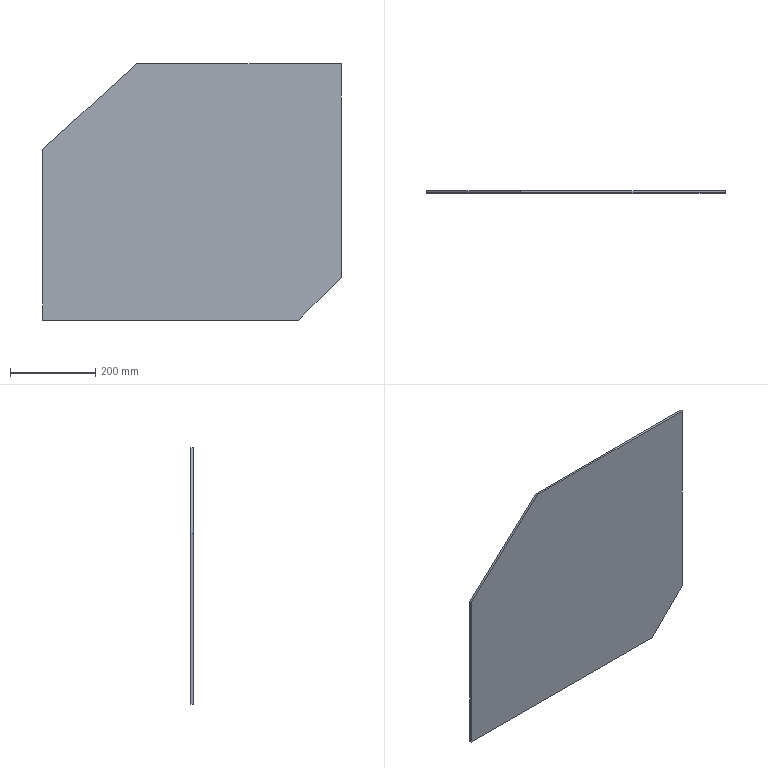Component | NX | CACANBA_2 | 1 solid | 8 faces | box 700 x 5 x 600 mm | volume 1965000 mm3 | plane 8
STEP:
#1=CARTESIAN_POINT('',(0.,0.,0.));
#2=DIRECTION('',(0.,0.,1.));
#3=DIRECTION('',(1.,0.,0.));
#4=AXIS2_PLACEMENT_3D('',#1,#2,#3);
#5=CARTESIAN_POINT('',(-10.,765.233,680.));
#6=VERTEX_POINT('',#5);
#7=CARTESIAN_POINT('',(-10.,765.233,180.));
#8=VERTEX_POINT('',#7);
#9=CARTESIAN_POINT('',(-10.,765.233,680.));
#10=DIRECTION('',(-0.,0.,-1.));
#11=VECTOR('',#10,1.);
#12=LINE('',#9,#11);
#13=CARTESIAN_POINT('',(-10.,770.233,680.));
#14=DIRECTION('',(-1.,0.,0.));
#15=DIRECTION('',(-0.,0.,-1.));
#16=AXIS2_PLACEMENT_3D('',#13,#14,#15);
#17=PLANE('',#16);
#18=CARTESIAN_POINT('',(0.,5.));
#19=DIRECTION('',(1.,0.));
#20=VECTOR('',#19,1.);
#21=LINE('',#18,#20);
#22=(GEOMETRIC_REPRESENTATION_CONTEXT(2)PARAMETRIC_REPRESENTATION_CONTEXT()REPRESENTATION_CONTEXT('',''));
#23=DEFINITIONAL_REPRESENTATION('',(#21),#22);
#24=PCURVE('',#17,#23);
#25=CARTESIAN_POINT('',(-10.,765.233,80.));
#26=DIRECTION('',(0.,1.,0.));
#27=DIRECTION('',(0.,0.,-1.));
#28=AXIS2_PLACEMENT_3D('',#25,#26,#27);
#29=PLANE('',#28);
#30=CARTESIAN_POINT('',(-600.,-0.));
#31=DIRECTION('',(1.,0.));
#32=VECTOR('',#31,1.);
#33=LINE('',#30,#32);
#34=(GEOMETRIC_REPRESENTATION_CONTEXT(2)PARAMETRIC_REPRESENTATION_CONTEXT()REPRESENTATION_CONTEXT('',''));
#35=DEFINITIONAL_REPRESENTATION('',(#33),#34);
#36=PCURVE('',#29,#35);
#37=SURFACE_CURVE('',#12,(#24,#36),.PCURVE_S1.);
#38=EDGE_CURVE('',#6,#8,#37,.T.);
#39=ORIENTED_EDGE('',*,*,#38,.T.);
#40=CARTESIAN_POINT('',(-10.,770.233,180.));
#41=VERTEX_POINT('',#40);
#42=CARTESIAN_POINT('',(-10.,770.233,180.));
#43=DIRECTION('',(0.,-1.,0.));
#44=VECTOR('',#43,1.);
#45=LINE('',#42,#44);
#46=CARTESIAN_POINT('',(500.,0.));
#47=DIRECTION('',(0.,1.));
#48=VECTOR('',#47,1.);
#49=LINE('',#46,#48);
#50=(GEOMETRIC_REPRESENTATION_CONTEXT(2)PARAMETRIC_REPRESENTATION_CONTEXT()REPRESENTATION_CONTEXT('',''));
#51=DEFINITIONAL_REPRESENTATION('',(#49),#50);
#52=PCURVE('',#17,#51);
#53=CARTESIAN_POINT('',(-10.,770.233,180.));
#54=DIRECTION('',(-0.7071,0.,0.7071));
#55=DIRECTION('',(-0.7071,0.,-0.7071));
#56=AXIS2_PLACEMENT_3D('',#53,#54,#55);
#57=PLANE('',#56);
#58=CARTESIAN_POINT('',(0.,0.));
#59=DIRECTION('',(0.,1.));
#60=VECTOR('',#59,1.);
#61=LINE('',#58,#60);
#62=(GEOMETRIC_REPRESENTATION_CONTEXT(2)PARAMETRIC_REPRESENTATION_CONTEXT()REPRESENTATION_CONTEXT('',''));
#63=DEFINITIONAL_REPRESENTATION('',(#61),#62);
#64=PCURVE('',#57,#63);
#65=SURFACE_CURVE('',#45,(#52,#64),.PCURVE_S1.);
#66=EDGE_CURVE('',#41,#8,#65,.T.);
#67=ORIENTED_EDGE('',*,*,#66,.F.);
#68=CARTESIAN_POINT('',(-10.,770.233,680.));
#69=VERTEX_POINT('',#68);
#70=CARTESIAN_POINT('',(-10.,770.233,680.));
#71=DIRECTION('',(-0.,0.,-1.));
#72=VECTOR('',#71,1.);
#73=LINE('',#70,#72);
#74=CARTESIAN_POINT('',(0.,0.));
#75=DIRECTION('',(1.,0.));
#76=VECTOR('',#75,1.);
#77=LINE('',#74,#76);
#78=(GEOMETRIC_REPRESENTATION_CONTEXT(2)PARAMETRIC_REPRESENTATION_CONTEXT()REPRESENTATION_CONTEXT('',''));
#79=DEFINITIONAL_REPRESENTATION('',(#77),#78);
#80=PCURVE('',#17,#79);
#81=CARTESIAN_POINT('',(-10.,770.233,80.));
#82=DIRECTION('',(0.,1.,0.));
#83=DIRECTION('',(0.,0.,-1.));
#84=AXIS2_PLACEMENT_3D('',#81,#82,#83);
#85=PLANE('',#84);
#86=CARTESIAN_POINT('',(-600.,-0.));
#87=DIRECTION('',(1.,0.));
#88=VECTOR('',#87,1.);
#89=LINE('',#86,#88);
#90=(GEOMETRIC_REPRESENTATION_CONTEXT(2)PARAMETRIC_REPRESENTATION_CONTEXT()REPRESENTATION_CONTEXT('',''));
#91=DEFINITIONAL_REPRESENTATION('',(#89),#90);
#92=PCURVE('',#85,#91);
#93=SURFACE_CURVE('',#73,(#80,#92),.PCURVE_S1.);
#94=EDGE_CURVE('',#69,#41,#93,.T.);
#95=ORIENTED_EDGE('',*,*,#94,.F.);
#96=CARTESIAN_POINT('',(-10.,770.233,680.));
#97=DIRECTION('',(0.,-1.,0.));
#98=VECTOR('',#97,1.);
#99=LINE('',#96,#98);
#100=CARTESIAN_POINT('',(0.,0.));
#101=DIRECTION('',(0.,1.));
#102=VECTOR('',#101,1.);
#103=LINE('',#100,#102);
#104=(GEOMETRIC_REPRESENTATION_CONTEXT(2)PARAMETRIC_REPRESENTATION_CONTEXT()REPRESENTATION_CONTEXT('',''));
#105=DEFINITIONAL_REPRESENTATION('',(#103),#104);
#106=PCURVE('',#17,#105);
#107=CARTESIAN_POINT('',(-490.,770.233,680.));
#108=DIRECTION('',(-0.,0.,-1.));
#109=DIRECTION('',(1.,0.,-0.));
#110=AXIS2_PLACEMENT_3D('',#107,#108,#109);
#111=PLANE('',#110);
#112=CARTESIAN_POINT('',(480.,0.));
#113=DIRECTION('',(0.,1.));
#114=VECTOR('',#113,1.);
#115=LINE('',#112,#114);
#116=(GEOMETRIC_REPRESENTATION_CONTEXT(2)PARAMETRIC_REPRESENTATION_CONTEXT()REPRESENTATION_CONTEXT('',''));
#117=DEFINITIONAL_REPRESENTATION('',(#115),#116);
#118=PCURVE('',#111,#117);
#119=SURFACE_CURVE('',#99,(#106,#118),.PCURVE_S1.);
#120=EDGE_CURVE('',#69,#6,#119,.T.);
#121=ORIENTED_EDGE('',*,*,#120,.T.);
#122=EDGE_LOOP('',(#39,#67,#95,#121));
#123=FACE_BOUND('',#122,.T.);
#124=ADVANCED_FACE('',(#123),#17,.F.);
#125=CARTESIAN_POINT('',(-110.,765.233,80.));
#126=VERTEX_POINT('',#125);
#127=CARTESIAN_POINT('',(-10.,765.233,180.));
#128=DIRECTION('',(-0.7071,0.,-0.7071));
#129=VECTOR('',#128,1.);
#130=LINE('',#127,#129);
#131=CARTESIAN_POINT('',(0.,5.));
#132=DIRECTION('',(1.,0.));
#133=VECTOR('',#132,1.);
#134=LINE('',#131,#133);
#135=(GEOMETRIC_REPRESENTATION_CONTEXT(2)PARAMETRIC_REPRESENTATION_CONTEXT()REPRESENTATION_CONTEXT('',''));
#136=DEFINITIONAL_REPRESENTATION('',(#134),#135);
#137=PCURVE('',#57,#136);
#138=CARTESIAN_POINT('',(-100.,0.));
#139=DIRECTION('',(0.7071,0.7071));
#140=VECTOR('',#139,1.);
#141=LINE('',#138,#140);
#142=(GEOMETRIC_REPRESENTATION_CONTEXT(2)PARAMETRIC_REPRESENTATION_CONTEXT()REPRESENTATION_CONTEXT('',''));
#143=DEFINITIONAL_REPRESENTATION('',(#141),#142);
#144=PCURVE('',#29,#143);
#145=SURFACE_CURVE('',#130,(#137,#144),.PCURVE_S1.);
#146=EDGE_CURVE('',#8,#126,#145,.T.);
#147=ORIENTED_EDGE('',*,*,#146,.T.);
#148=CARTESIAN_POINT('',(-110.,770.233,80.));
#149=VERTEX_POINT('',#148);
#150=CARTESIAN_POINT('',(-110.,770.233,80.));
#151=DIRECTION('',(0.,-1.,0.));
#152=VECTOR('',#151,1.);
#153=LINE('',#150,#152);
#154=CARTESIAN_POINT('',(141.421,0.));
#155=DIRECTION('',(0.,1.));
#156=VECTOR('',#155,1.);
#157=LINE('',#154,#156);
#158=(GEOMETRIC_REPRESENTATION_CONTEXT(2)PARAMETRIC_REPRESENTATION_CONTEXT()REPRESENTATION_CONTEXT('',''));
#159=DEFINITIONAL_REPRESENTATION('',(#157),#158);
#160=PCURVE('',#57,#159);
#161=CARTESIAN_POINT('',(-110.,770.233,80.));
#162=DIRECTION('',(0.,0.,1.));
#163=DIRECTION('',(-1.,0.,0.));
#164=AXIS2_PLACEMENT_3D('',#161,#162,#163);
#165=PLANE('',#164);
#166=CARTESIAN_POINT('',(0.,0.));
#167=DIRECTION('',(0.,1.));
#168=VECTOR('',#167,1.);
#169=LINE('',#166,#168);
#170=(GEOMETRIC_REPRESENTATION_CONTEXT(2)PARAMETRIC_REPRESENTATION_CONTEXT()REPRESENTATION_CONTEXT('',''));
#171=DEFINITIONAL_REPRESENTATION('',(#169),#170);
#172=PCURVE('',#165,#171);
#173=SURFACE_CURVE('',#153,(#160,#172),.PCURVE_S1.);
#174=EDGE_CURVE('',#149,#126,#173,.T.);
#175=ORIENTED_EDGE('',*,*,#174,.F.);
#176=CARTESIAN_POINT('',(-10.,770.233,180.));
#177=DIRECTION('',(-0.7071,0.,-0.7071));
#178=VECTOR('',#177,1.);
#179=LINE('',#176,#178);
#180=CARTESIAN_POINT('',(0.,0.));
#181=DIRECTION('',(1.,0.));
#182=VECTOR('',#181,1.);
#183=LINE('',#180,#182);
#184=(GEOMETRIC_REPRESENTATION_CONTEXT(2)PARAMETRIC_REPRESENTATION_CONTEXT()REPRESENTATION_CONTEXT('',''));
#185=DEFINITIONAL_REPRESENTATION('',(#183),#184);
#186=PCURVE('',#57,#185);
#187=CARTESIAN_POINT('',(-100.,0.));
#188=DIRECTION('',(0.7071,0.7071));
#189=VECTOR('',#188,1.);
#190=LINE('',#187,#189);
#191=(GEOMETRIC_REPRESENTATION_CONTEXT(2)PARAMETRIC_REPRESENTATION_CONTEXT()REPRESENTATION_CONTEXT('',''));
#192=DEFINITIONAL_REPRESENTATION('',(#190),#191);
#193=PCURVE('',#85,#192);
#194=SURFACE_CURVE('',#179,(#186,#193),.PCURVE_S1.);
#195=EDGE_CURVE('',#41,#149,#194,.T.);
#196=ORIENTED_EDGE('',*,*,#195,.F.);
#197=ORIENTED_EDGE('',*,*,#66,.T.);
#198=EDGE_LOOP('',(#147,#175,#196,#197));
#199=FACE_BOUND('',#198,.T.);
#200=ADVANCED_FACE('',(#199),#57,.F.);
#201=CARTESIAN_POINT('',(-710.,765.233,80.));
#202=VERTEX_POINT('',#201);
#203=CARTESIAN_POINT('',(-110.,765.233,80.));
#204=DIRECTION('',(-1.,0.,0.));
#205=VECTOR('',#204,1.);
#206=LINE('',#203,#205);
#207=CARTESIAN_POINT('',(0.,5.));
#208=DIRECTION('',(1.,0.));
#209=VECTOR('',#208,1.);
#210=LINE('',#207,#209);
#211=(GEOMETRIC_REPRESENTATION_CONTEXT(2)PARAMETRIC_REPRESENTATION_CONTEXT()REPRESENTATION_CONTEXT('',''));
#212=DEFINITIONAL_REPRESENTATION('',(#210),#211);
#213=PCURVE('',#165,#212);
#214=CARTESIAN_POINT('',(0.,100.));
#215=DIRECTION('',(-0.,1.));
#216=VECTOR('',#215,1.);
#217=LINE('',#214,#216);
#218=(GEOMETRIC_REPRESENTATION_CONTEXT(2)PARAMETRIC_REPRESENTATION_CONTEXT()REPRESENTATION_CONTEXT('',''));
#219=DEFINITIONAL_REPRESENTATION('',(#217),#218);
#220=PCURVE('',#29,#219);
#221=SURFACE_CURVE('',#206,(#213,#220),.PCURVE_S1.);
#222=EDGE_CURVE('',#126,#202,#221,.T.);
#223=ORIENTED_EDGE('',*,*,#222,.T.);
#224=CARTESIAN_POINT('',(-710.,770.233,80.));
#225=VERTEX_POINT('',#224);
#226=CARTESIAN_POINT('',(-710.,770.233,80.));
#227=DIRECTION('',(0.,-1.,0.));
#228=VECTOR('',#227,1.);
#229=LINE('',#226,#228);
#230=CARTESIAN_POINT('',(600.,0.));
#231=DIRECTION('',(0.,1.));
#232=VECTOR('',#231,1.);
#233=LINE('',#230,#232);
#234=(GEOMETRIC_REPRESENTATION_CONTEXT(2)PARAMETRIC_REPRESENTATION_CONTEXT()REPRESENTATION_CONTEXT('',''));
#235=DEFINITIONAL_REPRESENTATION('',(#233),#234);
#236=PCURVE('',#165,#235);
#237=CARTESIAN_POINT('',(-710.,770.233,80.));
#238=DIRECTION('',(1.,0.,-0.));
#239=DIRECTION('',(0.,0.,1.));
#240=AXIS2_PLACEMENT_3D('',#237,#238,#239);
#241=PLANE('',#240);
#242=CARTESIAN_POINT('',(0.,0.));
#243=DIRECTION('',(0.,1.));
#244=VECTOR('',#243,1.);
#245=LINE('',#242,#244);
#246=(GEOMETRIC_REPRESENTATION_CONTEXT(2)PARAMETRIC_REPRESENTATION_CONTEXT()REPRESENTATION_CONTEXT('',''));
#247=DEFINITIONAL_REPRESENTATION('',(#245),#246);
#248=PCURVE('',#241,#247);
#249=SURFACE_CURVE('',#229,(#236,#248),.PCURVE_S1.);
#250=EDGE_CURVE('',#225,#202,#249,.T.);
#251=ORIENTED_EDGE('',*,*,#250,.F.);
#252=CARTESIAN_POINT('',(-110.,770.233,80.));
#253=DIRECTION('',(-1.,0.,0.));
#254=VECTOR('',#253,1.);
#255=LINE('',#252,#254);
#256=CARTESIAN_POINT('',(0.,0.));
#257=DIRECTION('',(1.,0.));
#258=VECTOR('',#257,1.);
#259=LINE('',#256,#258);
#260=(GEOMETRIC_REPRESENTATION_CONTEXT(2)PARAMETRIC_REPRESENTATION_CONTEXT()REPRESENTATION_CONTEXT('',''));
#261=DEFINITIONAL_REPRESENTATION('',(#259),#260);
#262=PCURVE('',#165,#261);
#263=CARTESIAN_POINT('',(0.,100.));
#264=DIRECTION('',(-0.,1.));
#265=VECTOR('',#264,1.);
#266=LINE('',#263,#265);
#267=(GEOMETRIC_REPRESENTATION_CONTEXT(2)PARAMETRIC_REPRESENTATION_CONTEXT()REPRESENTATION_CONTEXT('',''));
#268=DEFINITIONAL_REPRESENTATION('',(#266),#267);
#269=PCURVE('',#85,#268);
#270=SURFACE_CURVE('',#255,(#262,#269),.PCURVE_S1.);
#271=EDGE_CURVE('',#149,#225,#270,.T.);
#272=ORIENTED_EDGE('',*,*,#271,.F.);
#273=ORIENTED_EDGE('',*,*,#174,.T.);
#274=EDGE_LOOP('',(#223,#251,#272,#273));
#275=FACE_BOUND('',#274,.T.);
#276=ADVANCED_FACE('',(#275),#165,.F.);
#277=CARTESIAN_POINT('',(-710.,765.233,480.));
#278=VERTEX_POINT('',#277);
#279=CARTESIAN_POINT('',(-710.,765.233,80.));
#280=DIRECTION('',(0.,0.,1.));
#281=VECTOR('',#280,1.);
#282=LINE('',#279,#281);
#283=CARTESIAN_POINT('',(0.,5.));
#284=DIRECTION('',(1.,0.));
#285=VECTOR('',#284,1.);
#286=LINE('',#283,#285);
#287=(GEOMETRIC_REPRESENTATION_CONTEXT(2)PARAMETRIC_REPRESENTATION_CONTEXT()REPRESENTATION_CONTEXT('',''));
#288=DEFINITIONAL_REPRESENTATION('',(#286),#287);
#289=PCURVE('',#241,#288);
#290=CARTESIAN_POINT('',(-0.,700.));
#291=DIRECTION('',(-1.,-0.));
#292=VECTOR('',#291,1.);
#293=LINE('',#290,#292);
#294=(GEOMETRIC_REPRESENTATION_CONTEXT(2)PARAMETRIC_REPRESENTATION_CONTEXT()REPRESENTATION_CONTEXT('',''));
#295=DEFINITIONAL_REPRESENTATION('',(#293),#294);
#296=PCURVE('',#29,#295);
#297=SURFACE_CURVE('',#282,(#289,#296),.PCURVE_S1.);
#298=EDGE_CURVE('',#202,#278,#297,.T.);
#299=ORIENTED_EDGE('',*,*,#298,.T.);
#300=CARTESIAN_POINT('',(-710.,770.233,480.));
#301=VERTEX_POINT('',#300);
#302=CARTESIAN_POINT('',(-710.,770.233,480.));
#303=DIRECTION('',(0.,-1.,0.));
#304=VECTOR('',#303,1.);
#305=LINE('',#302,#304);
#306=CARTESIAN_POINT('',(400.,0.));
#307=DIRECTION('',(0.,1.));
#308=VECTOR('',#307,1.);
#309=LINE('',#306,#308);
#310=(GEOMETRIC_REPRESENTATION_CONTEXT(2)PARAMETRIC_REPRESENTATION_CONTEXT()REPRESENTATION_CONTEXT('',''));
#311=DEFINITIONAL_REPRESENTATION('',(#309),#310);
#312=PCURVE('',#241,#311);
#313=CARTESIAN_POINT('',(-710.,770.233,480.));
#314=DIRECTION('',(0.6727,0.,-0.7399));
#315=DIRECTION('',(0.7399,0.,0.6727));
#316=AXIS2_PLACEMENT_3D('',#313,#314,#315);
#317=PLANE('',#316);
#318=CARTESIAN_POINT('',(0.,0.));
#319=DIRECTION('',(0.,1.));
#320=VECTOR('',#319,1.);
#321=LINE('',#318,#320);
#322=(GEOMETRIC_REPRESENTATION_CONTEXT(2)PARAMETRIC_REPRESENTATION_CONTEXT()REPRESENTATION_CONTEXT('',''));
#323=DEFINITIONAL_REPRESENTATION('',(#321),#322);
#324=PCURVE('',#317,#323);
#325=SURFACE_CURVE('',#305,(#312,#324),.PCURVE_S1.);
#326=EDGE_CURVE('',#301,#278,#325,.T.);
#327=ORIENTED_EDGE('',*,*,#326,.F.);
#328=CARTESIAN_POINT('',(-710.,770.233,80.));
#329=DIRECTION('',(0.,0.,1.));
#330=VECTOR('',#329,1.);
#331=LINE('',#328,#330);
#332=CARTESIAN_POINT('',(0.,0.));
#333=DIRECTION('',(1.,0.));
#334=VECTOR('',#333,1.);
#335=LINE('',#332,#334);
#336=(GEOMETRIC_REPRESENTATION_CONTEXT(2)PARAMETRIC_REPRESENTATION_CONTEXT()REPRESENTATION_CONTEXT('',''));
#337=DEFINITIONAL_REPRESENTATION('',(#335),#336);
#338=PCURVE('',#241,#337);
#339=CARTESIAN_POINT('',(-0.,700.));
#340=DIRECTION('',(-1.,-0.));
#341=VECTOR('',#340,1.);
#342=LINE('',#339,#341);
#343=(GEOMETRIC_REPRESENTATION_CONTEXT(2)PARAMETRIC_REPRESENTATION_CONTEXT()REPRESENTATION_CONTEXT('',''));
#344=DEFINITIONAL_REPRESENTATION('',(#342),#343);
#345=PCURVE('',#85,#344);
#346=SURFACE_CURVE('',#331,(#338,#345),.PCURVE_S1.);
#347=EDGE_CURVE('',#225,#301,#346,.T.);
#348=ORIENTED_EDGE('',*,*,#347,.F.);
#349=ORIENTED_EDGE('',*,*,#250,.T.);
#350=EDGE_LOOP('',(#299,#327,#348,#349));
#351=FACE_BOUND('',#350,.T.);
#352=ADVANCED_FACE('',(#351),#241,.F.);
#353=CARTESIAN_POINT('',(-490.,765.233,680.));
#354=VERTEX_POINT('',#353);
#355=CARTESIAN_POINT('',(-710.,765.233,480.));
#356=DIRECTION('',(0.7399,0.,0.6727));
#357=VECTOR('',#356,1.);
#358=LINE('',#355,#357);
#359=CARTESIAN_POINT('',(0.,5.));
#360=DIRECTION('',(1.,0.));
#361=VECTOR('',#360,1.);
#362=LINE('',#359,#361);
#363=(GEOMETRIC_REPRESENTATION_CONTEXT(2)PARAMETRIC_REPRESENTATION_CONTEXT()REPRESENTATION_CONTEXT('',''));
#364=DEFINITIONAL_REPRESENTATION('',(#362),#363);
#365=PCURVE('',#317,#364);
#366=CARTESIAN_POINT('',(-400.,700.));
#367=DIRECTION('',(-0.6727,-0.7399));
#368=VECTOR('',#367,1.);
#369=LINE('',#366,#368);
#370=(GEOMETRIC_REPRESENTATION_CONTEXT(2)PARAMETRIC_REPRESENTATION_CONTEXT()REPRESENTATION_CONTEXT('',''));
#371=DEFINITIONAL_REPRESENTATION('',(#369),#370);
#372=PCURVE('',#29,#371);
#373=SURFACE_CURVE('',#358,(#365,#372),.PCURVE_S1.);
#374=EDGE_CURVE('',#278,#354,#373,.T.);
#375=ORIENTED_EDGE('',*,*,#374,.T.);
#376=CARTESIAN_POINT('',(-490.,770.233,680.));
#377=VERTEX_POINT('',#376);
#378=CARTESIAN_POINT('',(-490.,770.233,680.));
#379=DIRECTION('',(0.,-1.,0.));
#380=VECTOR('',#379,1.);
#381=LINE('',#378,#380);
#382=CARTESIAN_POINT('',(297.321,0.));
#383=DIRECTION('',(0.,1.));
#384=VECTOR('',#383,1.);
#385=LINE('',#382,#384);
#386=(GEOMETRIC_REPRESENTATION_CONTEXT(2)PARAMETRIC_REPRESENTATION_CONTEXT()REPRESENTATION_CONTEXT('',''));
#387=DEFINITIONAL_REPRESENTATION('',(#385),#386);
#388=PCURVE('',#317,#387);
#389=CARTESIAN_POINT('',(0.,0.));
#390=DIRECTION('',(0.,1.));
#391=VECTOR('',#390,1.);
#392=LINE('',#389,#391);
#393=(GEOMETRIC_REPRESENTATION_CONTEXT(2)PARAMETRIC_REPRESENTATION_CONTEXT()REPRESENTATION_CONTEXT('',''));
#394=DEFINITIONAL_REPRESENTATION('',(#392),#393);
#395=PCURVE('',#111,#394);
#396=SURFACE_CURVE('',#381,(#388,#395),.PCURVE_S1.);
#397=EDGE_CURVE('',#377,#354,#396,.T.);
#398=ORIENTED_EDGE('',*,*,#397,.F.);
#399=CARTESIAN_POINT('',(-710.,770.233,480.));
#400=DIRECTION('',(0.7399,0.,0.6727));
#401=VECTOR('',#400,1.);
#402=LINE('',#399,#401);
#403=CARTESIAN_POINT('',(0.,0.));
#404=DIRECTION('',(1.,0.));
#405=VECTOR('',#404,1.);
#406=LINE('',#403,#405);
#407=(GEOMETRIC_REPRESENTATION_CONTEXT(2)PARAMETRIC_REPRESENTATION_CONTEXT()REPRESENTATION_CONTEXT('',''));
#408=DEFINITIONAL_REPRESENTATION('',(#406),#407);
#409=PCURVE('',#317,#408);
#410=CARTESIAN_POINT('',(-400.,700.));
#411=DIRECTION('',(-0.6727,-0.7399));
#412=VECTOR('',#411,1.);
#413=LINE('',#410,#412);
#414=(GEOMETRIC_REPRESENTATION_CONTEXT(2)PARAMETRIC_REPRESENTATION_CONTEXT()REPRESENTATION_CONTEXT('',''));
#415=DEFINITIONAL_REPRESENTATION('',(#413),#414);
#416=PCURVE('',#85,#415);
#417=SURFACE_CURVE('',#402,(#409,#416),.PCURVE_S1.);
#418=EDGE_CURVE('',#301,#377,#417,.T.);
#419=ORIENTED_EDGE('',*,*,#418,.F.);
#420=ORIENTED_EDGE('',*,*,#326,.T.);
#421=EDGE_LOOP('',(#375,#398,#419,#420));
#422=FACE_BOUND('',#421,.T.);
#423=ADVANCED_FACE('',(#422),#317,.F.);
#424=CARTESIAN_POINT('',(-490.,765.233,680.));
#425=DIRECTION('',(1.,0.,-0.));
#426=VECTOR('',#425,1.);
#427=LINE('',#424,#426);
#428=CARTESIAN_POINT('',(0.,5.));
#429=DIRECTION('',(1.,0.));
#430=VECTOR('',#429,1.);
#431=LINE('',#428,#430);
#432=(GEOMETRIC_REPRESENTATION_CONTEXT(2)PARAMETRIC_REPRESENTATION_CONTEXT()REPRESENTATION_CONTEXT('',''));
#433=DEFINITIONAL_REPRESENTATION('',(#431),#432);
#434=PCURVE('',#111,#433);
#435=CARTESIAN_POINT('',(-600.,480.));
#436=DIRECTION('',(0.,-1.));
#437=VECTOR('',#436,1.);
#438=LINE('',#435,#437);
#439=(GEOMETRIC_REPRESENTATION_CONTEXT(2)PARAMETRIC_REPRESENTATION_CONTEXT()REPRESENTATION_CONTEXT('',''));
#440=DEFINITIONAL_REPRESENTATION('',(#438),#439);
#441=PCURVE('',#29,#440);
#442=SURFACE_CURVE('',#427,(#434,#441),.PCURVE_S1.);
#443=EDGE_CURVE('',#354,#6,#442,.T.);
#444=ORIENTED_EDGE('',*,*,#443,.T.);
#445=ORIENTED_EDGE('',*,*,#120,.F.);
#446=CARTESIAN_POINT('',(-490.,770.233,680.));
#447=DIRECTION('',(1.,0.,-0.));
#448=VECTOR('',#447,1.);
#449=LINE('',#446,#448);
#450=CARTESIAN_POINT('',(0.,0.));
#451=DIRECTION('',(1.,0.));
#452=VECTOR('',#451,1.);
#453=LINE('',#450,#452);
#454=(GEOMETRIC_REPRESENTATION_CONTEXT(2)PARAMETRIC_REPRESENTATION_CONTEXT()REPRESENTATION_CONTEXT('',''));
#455=DEFINITIONAL_REPRESENTATION('',(#453),#454);
#456=PCURVE('',#111,#455);
#457=CARTESIAN_POINT('',(-600.,480.));
#458=DIRECTION('',(0.,-1.));
#459=VECTOR('',#458,1.);
#460=LINE('',#457,#459);
#461=(GEOMETRIC_REPRESENTATION_CONTEXT(2)PARAMETRIC_REPRESENTATION_CONTEXT()REPRESENTATION_CONTEXT('',''));
#462=DEFINITIONAL_REPRESENTATION('',(#460),#461);
#463=PCURVE('',#85,#462);
#464=SURFACE_CURVE('',#449,(#456,#463),.PCURVE_S1.);
#465=EDGE_CURVE('',#377,#69,#464,.T.);
#466=ORIENTED_EDGE('',*,*,#465,.F.);
#467=ORIENTED_EDGE('',*,*,#397,.T.);
#468=EDGE_LOOP('',(#444,#445,#466,#467));
#469=FACE_BOUND('',#468,.T.);
#470=ADVANCED_FACE('',(#469),#111,.F.);
#471=ORIENTED_EDGE('',*,*,#94,.T.);
#472=ORIENTED_EDGE('',*,*,#195,.T.);
#473=ORIENTED_EDGE('',*,*,#271,.T.);
#474=ORIENTED_EDGE('',*,*,#347,.T.);
#475=ORIENTED_EDGE('',*,*,#418,.T.);
#476=ORIENTED_EDGE('',*,*,#465,.T.);
#477=EDGE_LOOP('',(#471,#472,#473,#474,#475,#476));
#478=FACE_BOUND('',#477,.T.);
#479=ADVANCED_FACE('',(#478),#85,.T.);
#480=ORIENTED_EDGE('',*,*,#38,.F.);
#481=ORIENTED_EDGE('',*,*,#443,.F.);
#482=ORIENTED_EDGE('',*,*,#374,.F.);
#483=ORIENTED_EDGE('',*,*,#298,.F.);
#484=ORIENTED_EDGE('',*,*,#222,.F.);
#485=ORIENTED_EDGE('',*,*,#146,.F.);
#486=EDGE_LOOP('',(#480,#481,#482,#483,#484,#485));
#487=FACE_BOUND('',#486,.T.);
#488=ADVANCED_FACE('',(#487),#29,.F.);
#489=CLOSED_SHELL('',(#124,#200,#276,#352,#423,#470,#479,#488));
#490=MANIFOLD_SOLID_BREP('',#489);
#491=(LENGTH_UNIT()NAMED_UNIT(*)SI_UNIT(.MILLI.,.METRE.));
#492=UNCERTAINTY_MEASURE_WITH_UNIT(LENGTH_MEASURE(0.0000001),#491,'','');
#493=(NAMED_UNIT(*)PLANE_ANGLE_UNIT()SI_UNIT($,.RADIAN.));
#494=(NAMED_UNIT(*)SI_UNIT($,.STERADIAN.)SOLID_ANGLE_UNIT());
#495=(GEOMETRIC_REPRESENTATION_CONTEXT(3)GLOBAL_UNCERTAINTY_ASSIGNED_CONTEXT((#492))GLOBAL_UNIT_ASSIGNED_CONTEXT((#491,#493,#494))REPRESENTATION_CONTEXT('',''));
#496=ADVANCED_BREP_SHAPE_REPRESENTATION('',(#4,#490),#495);